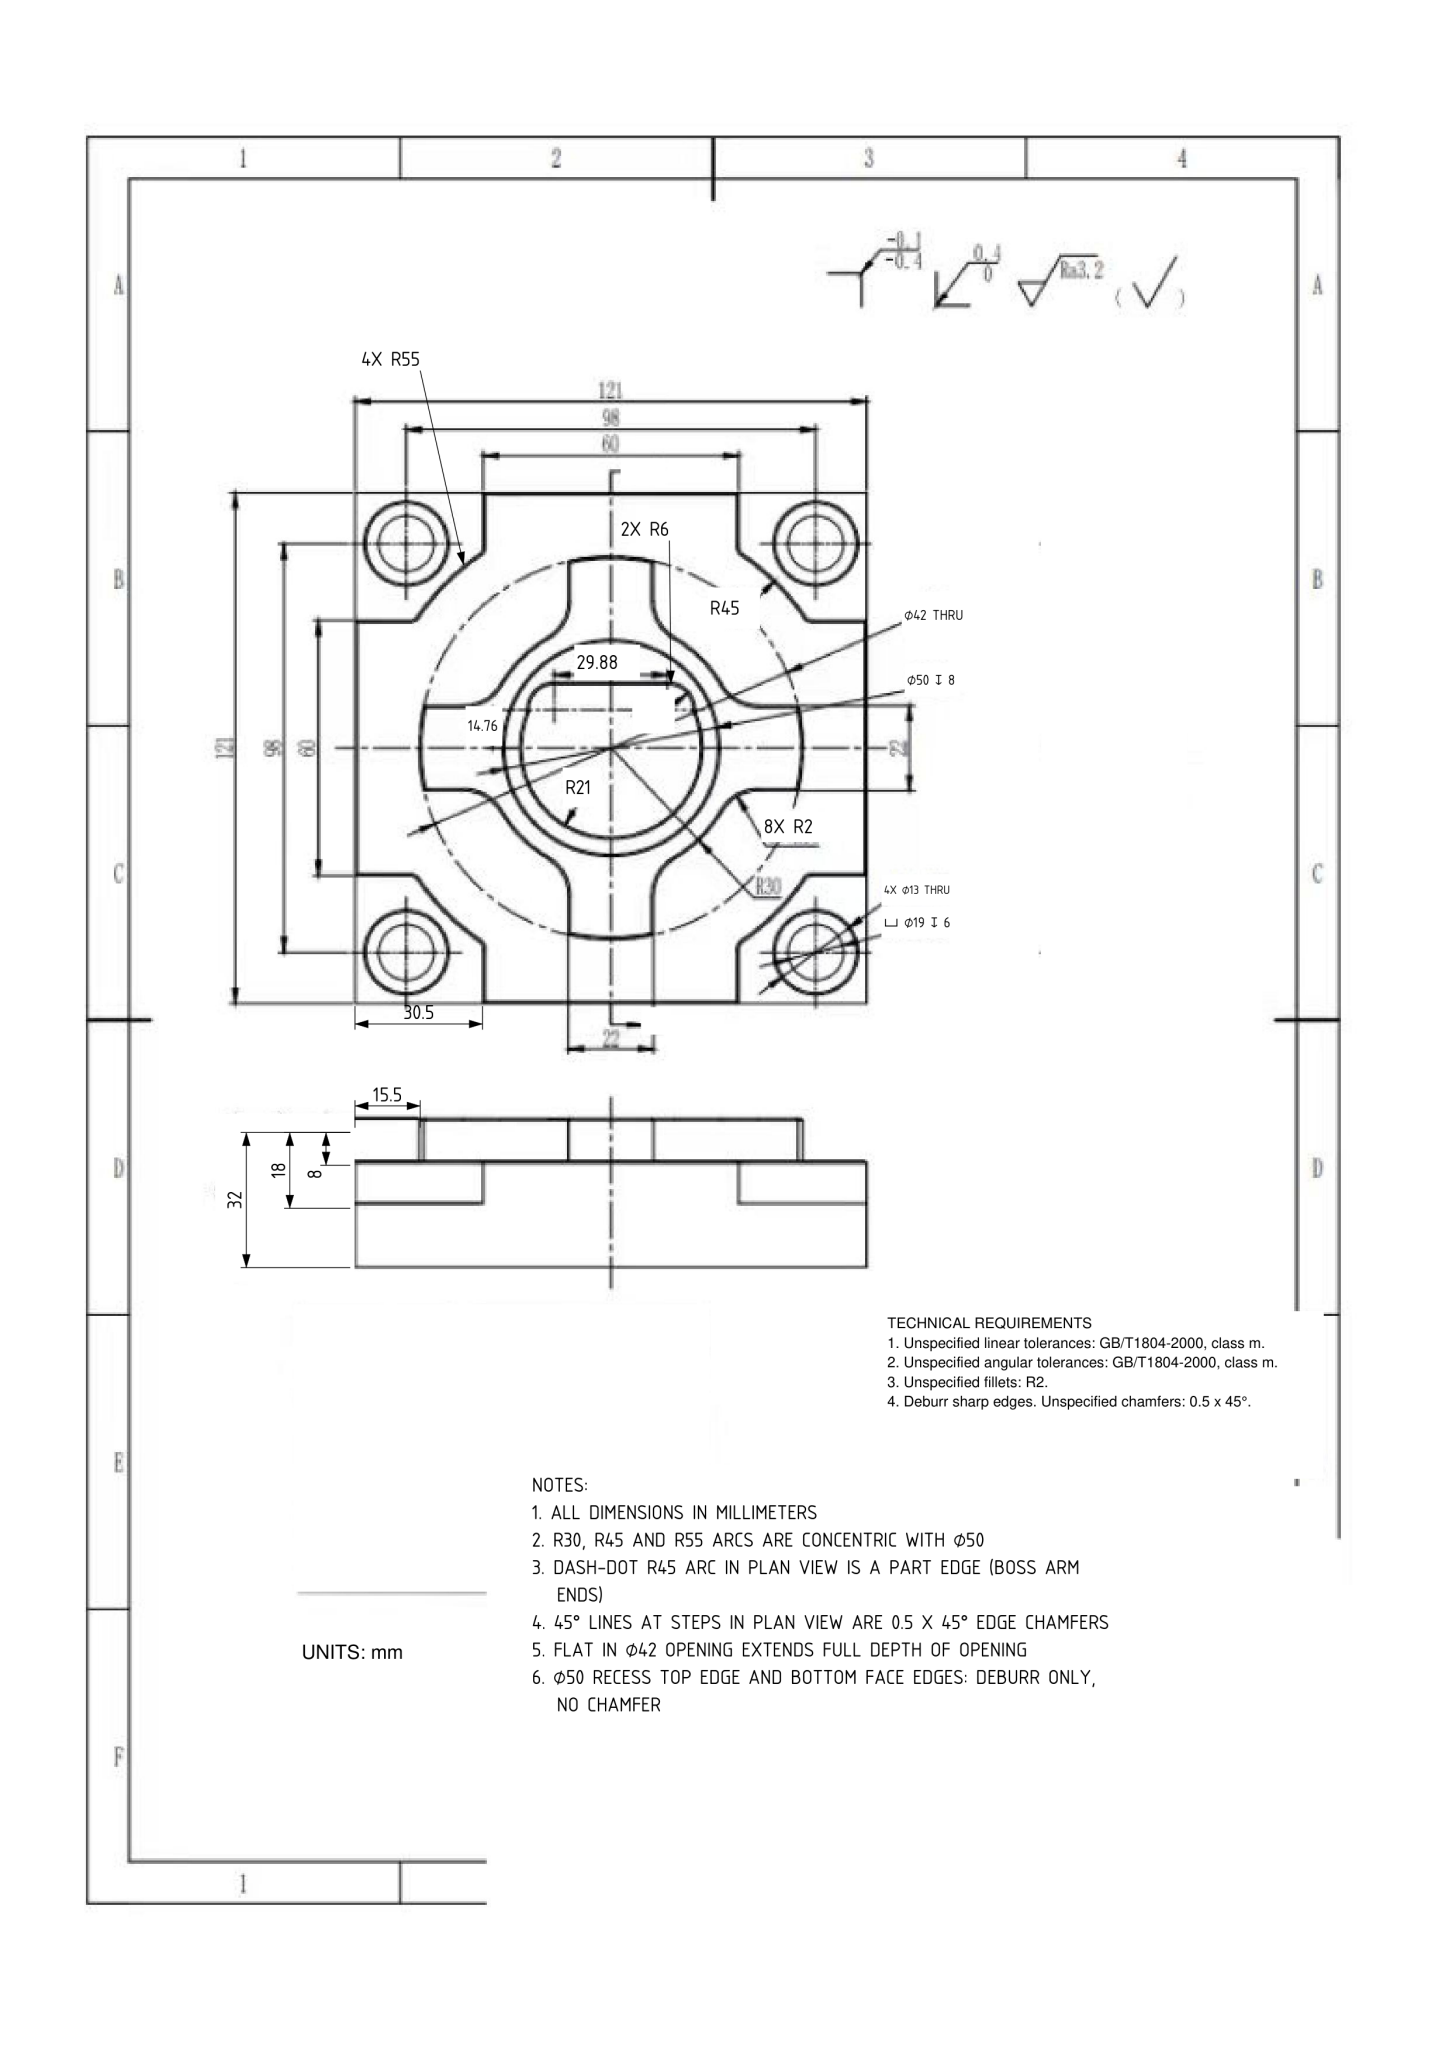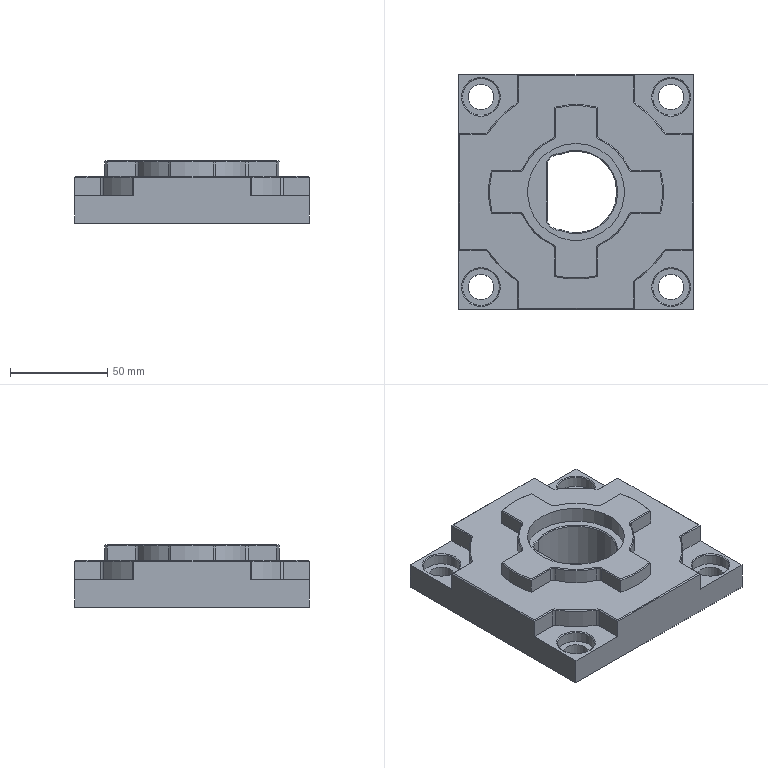Part | NX | mm | 1 solid | 129 faces | box 121 x 121 x 32 mm | volume 296138 mm3 | plane 54 | cylinder 40 | cone 35 | commonest cylinder face diameters 4 x16 110 x4 90 x4 60 x4 13 x4 19 x4 12 x2 50 x1